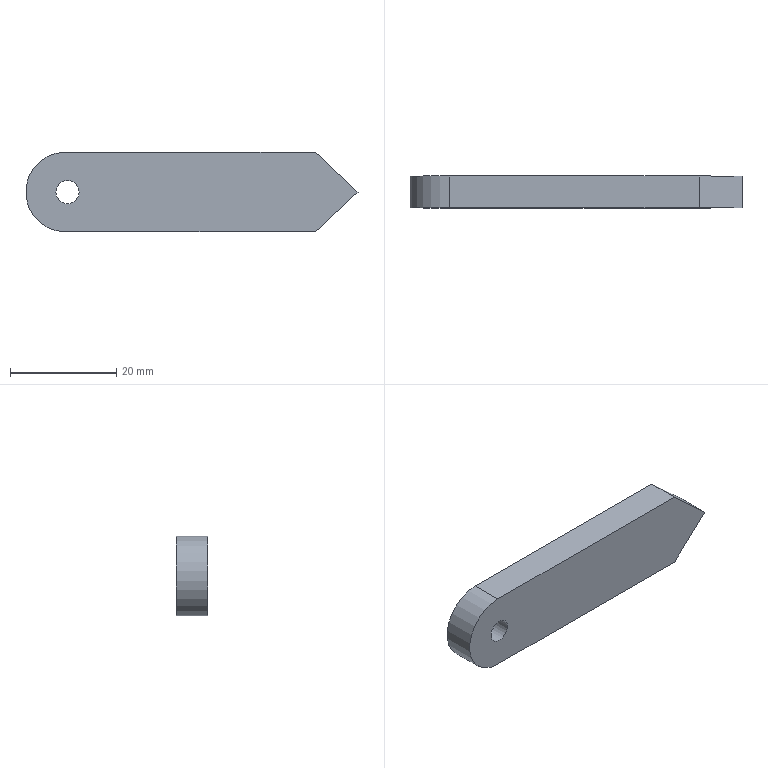Component | NX | TRI_SLIDER_2 | 1 solid | 8 faces | box 62.5 x 6 x 15 mm | volume 5028 mm3 | plane 6 | cylinder 2 | commonest cylinder face diameters 15 x1 4.371 x1
STEP:
#1=CARTESIAN_POINT('',(0.,0.,0.));
#2=DIRECTION('',(0.,0.,1.));
#3=DIRECTION('',(1.,0.,0.));
#4=AXIS2_PLACEMENT_3D('',#1,#2,#3);
#5=CARTESIAN_POINT('',(53.887,-12.,79.479));
#6=VERTEX_POINT('',#5);
#7=CARTESIAN_POINT('',(45.867,-12.,72.));
#8=VERTEX_POINT('',#7);
#9=CARTESIAN_POINT('',(53.887,-12.,79.479));
#10=DIRECTION('',(-0.7314,0.,-0.682));
#11=VECTOR('',#10,1.);
#12=LINE('',#9,#11);
#13=CARTESIAN_POINT('',(53.887,-18.,79.479));
#14=DIRECTION('',(0.682,0.,-0.7314));
#15=DIRECTION('',(0.7314,0.,0.682));
#16=AXIS2_PLACEMENT_3D('',#13,#14,#15);
#17=PLANE('',#16);
#18=CARTESIAN_POINT('',(0.,-6.));
#19=DIRECTION('',(-1.,0.));
#20=VECTOR('',#19,1.);
#21=LINE('',#18,#20);
#22=(GEOMETRIC_REPRESENTATION_CONTEXT(2)PARAMETRIC_REPRESENTATION_CONTEXT()REPRESENTATION_CONTEXT('',''));
#23=DEFINITIONAL_REPRESENTATION('',(#21),#22);
#24=PCURVE('',#17,#23);
#25=CARTESIAN_POINT('',(-1.113,-12.,79.5));
#26=DIRECTION('',(0.,1.,0.));
#27=DIRECTION('',(1.,0.,0.));
#28=AXIS2_PLACEMENT_3D('',#25,#26,#27);
#29=PLANE('',#28);
#30=CARTESIAN_POINT('',(55.,0.02132));
#31=DIRECTION('',(-0.7314,0.682));
#32=VECTOR('',#31,1.);
#33=LINE('',#30,#32);
#34=(GEOMETRIC_REPRESENTATION_CONTEXT(2)PARAMETRIC_REPRESENTATION_CONTEXT()REPRESENTATION_CONTEXT('',''));
#35=DEFINITIONAL_REPRESENTATION('',(#33),#34);
#36=PCURVE('',#29,#35);
#37=SURFACE_CURVE('',#12,(#24,#36),.PCURVE_S1.);
#38=EDGE_CURVE('',#6,#8,#37,.T.);
#39=ORIENTED_EDGE('',*,*,#38,.F.);
#40=CARTESIAN_POINT('',(53.887,-18.,79.479));
#41=VERTEX_POINT('',#40);
#42=CARTESIAN_POINT('',(53.887,-18.,79.479));
#43=DIRECTION('',(0.,1.,0.));
#44=VECTOR('',#43,1.);
#45=LINE('',#42,#44);
#46=CARTESIAN_POINT('',(0.,0.));
#47=DIRECTION('',(0.,-1.));
#48=VECTOR('',#47,1.);
#49=LINE('',#46,#48);
#50=(GEOMETRIC_REPRESENTATION_CONTEXT(2)PARAMETRIC_REPRESENTATION_CONTEXT()REPRESENTATION_CONTEXT('',''));
#51=DEFINITIONAL_REPRESENTATION('',(#49),#50);
#52=PCURVE('',#17,#51);
#53=CARTESIAN_POINT('',(45.822,-18.,87.));
#54=DIRECTION('',(0.682,0.,0.7314));
#55=DIRECTION('',(-0.7314,0.,0.682));
#56=AXIS2_PLACEMENT_3D('',#53,#54,#55);
#57=PLANE('',#56);
#58=CARTESIAN_POINT('',(-11.028,0.));
#59=DIRECTION('',(0.,-1.));
#60=VECTOR('',#59,1.);
#61=LINE('',#58,#60);
#62=(GEOMETRIC_REPRESENTATION_CONTEXT(2)PARAMETRIC_REPRESENTATION_CONTEXT()REPRESENTATION_CONTEXT('',''));
#63=DEFINITIONAL_REPRESENTATION('',(#61),#62);
#64=PCURVE('',#57,#63);
#65=SURFACE_CURVE('',#45,(#52,#64),.PCURVE_S1.);
#66=EDGE_CURVE('',#41,#6,#65,.T.);
#67=ORIENTED_EDGE('',*,*,#66,.F.);
#68=CARTESIAN_POINT('',(45.867,-18.,72.));
#69=VERTEX_POINT('',#68);
#70=CARTESIAN_POINT('',(53.887,-18.,79.479));
#71=DIRECTION('',(-0.7314,0.,-0.682));
#72=VECTOR('',#71,1.);
#73=LINE('',#70,#72);
#74=CARTESIAN_POINT('',(0.,0.));
#75=DIRECTION('',(-1.,0.));
#76=VECTOR('',#75,1.);
#77=LINE('',#74,#76);
#78=(GEOMETRIC_REPRESENTATION_CONTEXT(2)PARAMETRIC_REPRESENTATION_CONTEXT()REPRESENTATION_CONTEXT('',''));
#79=DEFINITIONAL_REPRESENTATION('',(#77),#78);
#80=PCURVE('',#17,#79);
#81=CARTESIAN_POINT('',(-1.113,-18.,79.5));
#82=DIRECTION('',(0.,1.,0.));
#83=DIRECTION('',(1.,0.,0.));
#84=AXIS2_PLACEMENT_3D('',#81,#82,#83);
#85=PLANE('',#84);
#86=CARTESIAN_POINT('',(55.,0.02132));
#87=DIRECTION('',(-0.7314,0.682));
#88=VECTOR('',#87,1.);
#89=LINE('',#86,#88);
#90=(GEOMETRIC_REPRESENTATION_CONTEXT(2)PARAMETRIC_REPRESENTATION_CONTEXT()REPRESENTATION_CONTEXT('',''));
#91=DEFINITIONAL_REPRESENTATION('',(#89),#90);
#92=PCURVE('',#85,#91);
#93=SURFACE_CURVE('',#73,(#80,#92),.PCURVE_S1.);
#94=EDGE_CURVE('',#41,#69,#93,.T.);
#95=ORIENTED_EDGE('',*,*,#94,.T.);
#96=CARTESIAN_POINT('',(45.867,-18.,72.));
#97=DIRECTION('',(0.,1.,0.));
#98=VECTOR('',#97,1.);
#99=LINE('',#96,#98);
#100=CARTESIAN_POINT('',(-10.966,0.));
#101=DIRECTION('',(0.,-1.));
#102=VECTOR('',#101,1.);
#103=LINE('',#100,#102);
#104=(GEOMETRIC_REPRESENTATION_CONTEXT(2)PARAMETRIC_REPRESENTATION_CONTEXT()REPRESENTATION_CONTEXT('',''));
#105=DEFINITIONAL_REPRESENTATION('',(#103),#104);
#106=PCURVE('',#17,#105);
#107=CARTESIAN_POINT('',(45.867,-18.,72.));
#108=DIRECTION('',(0.,0.,-1.));
#109=DIRECTION('',(1.,0.,0.));
#110=AXIS2_PLACEMENT_3D('',#107,#108,#109);
#111=PLANE('',#110);
#112=CARTESIAN_POINT('',(0.,0.));
#113=DIRECTION('',(0.,-1.));
#114=VECTOR('',#113,1.);
#115=LINE('',#112,#114);
#116=(GEOMETRIC_REPRESENTATION_CONTEXT(2)PARAMETRIC_REPRESENTATION_CONTEXT()REPRESENTATION_CONTEXT('',''));
#117=DEFINITIONAL_REPRESENTATION('',(#115),#116);
#118=PCURVE('',#111,#117);
#119=SURFACE_CURVE('',#99,(#106,#118),.PCURVE_S1.);
#120=EDGE_CURVE('',#69,#8,#119,.T.);
#121=ORIENTED_EDGE('',*,*,#120,.T.);
#122=EDGE_LOOP('',(#39,#67,#95,#121));
#123=FACE_BOUND('',#122,.T.);
#124=ADVANCED_FACE('',(#123),#17,.T.);
#125=CARTESIAN_POINT('',(-1.113,-12.,72.));
#126=VERTEX_POINT('',#125);
#127=CARTESIAN_POINT('',(45.867,-12.,72.));
#128=DIRECTION('',(-1.,0.,-0.));
#129=VECTOR('',#128,1.);
#130=LINE('',#127,#129);
#131=CARTESIAN_POINT('',(0.,-6.));
#132=DIRECTION('',(-1.,0.));
#133=VECTOR('',#132,1.);
#134=LINE('',#131,#133);
#135=(GEOMETRIC_REPRESENTATION_CONTEXT(2)PARAMETRIC_REPRESENTATION_CONTEXT()REPRESENTATION_CONTEXT('',''));
#136=DEFINITIONAL_REPRESENTATION('',(#134),#135);
#137=PCURVE('',#111,#136);
#138=CARTESIAN_POINT('',(46.98,7.5));
#139=DIRECTION('',(-1.,0.));
#140=VECTOR('',#139,1.);
#141=LINE('',#138,#140);
#142=(GEOMETRIC_REPRESENTATION_CONTEXT(2)PARAMETRIC_REPRESENTATION_CONTEXT()REPRESENTATION_CONTEXT('',''));
#143=DEFINITIONAL_REPRESENTATION('',(#141),#142);
#144=PCURVE('',#29,#143);
#145=SURFACE_CURVE('',#130,(#137,#144),.PCURVE_S1.);
#146=EDGE_CURVE('',#8,#126,#145,.T.);
#147=ORIENTED_EDGE('',*,*,#146,.F.);
#148=ORIENTED_EDGE('',*,*,#120,.F.);
#149=CARTESIAN_POINT('',(-1.113,-18.,72.));
#150=VERTEX_POINT('',#149);
#151=CARTESIAN_POINT('',(45.867,-18.,72.));
#152=DIRECTION('',(-1.,0.,-0.));
#153=VECTOR('',#152,1.);
#154=LINE('',#151,#153);
#155=CARTESIAN_POINT('',(0.,0.));
#156=DIRECTION('',(-1.,0.));
#157=VECTOR('',#156,1.);
#158=LINE('',#155,#157);
#159=(GEOMETRIC_REPRESENTATION_CONTEXT(2)PARAMETRIC_REPRESENTATION_CONTEXT()REPRESENTATION_CONTEXT('',''));
#160=DEFINITIONAL_REPRESENTATION('',(#158),#159);
#161=PCURVE('',#111,#160);
#162=CARTESIAN_POINT('',(46.98,7.5));
#163=DIRECTION('',(-1.,0.));
#164=VECTOR('',#163,1.);
#165=LINE('',#162,#164);
#166=(GEOMETRIC_REPRESENTATION_CONTEXT(2)PARAMETRIC_REPRESENTATION_CONTEXT()REPRESENTATION_CONTEXT('',''));
#167=DEFINITIONAL_REPRESENTATION('',(#165),#166);
#168=PCURVE('',#85,#167);
#169=SURFACE_CURVE('',#154,(#161,#168),.PCURVE_S1.);
#170=EDGE_CURVE('',#69,#150,#169,.T.);
#171=ORIENTED_EDGE('',*,*,#170,.T.);
#172=CARTESIAN_POINT('',(-1.113,-18.,72.));
#173=DIRECTION('',(0.,1.,0.));
#174=VECTOR('',#173,1.);
#175=LINE('',#172,#174);
#176=CARTESIAN_POINT('',(-46.98,0.));
#177=DIRECTION('',(0.,-1.));
#178=VECTOR('',#177,1.);
#179=LINE('',#176,#178);
#180=(GEOMETRIC_REPRESENTATION_CONTEXT(2)PARAMETRIC_REPRESENTATION_CONTEXT()REPRESENTATION_CONTEXT('',''));
#181=DEFINITIONAL_REPRESENTATION('',(#179),#180);
#182=PCURVE('',#111,#181);
#183=CARTESIAN_POINT('',(-1.113,-18.,79.5));
#184=DIRECTION('',(0.,1.,0.));
#185=DIRECTION('',(1.,0.,0.));
#186=AXIS2_PLACEMENT_3D('',#183,#184,#185);
#187=CYLINDRICAL_SURFACE('',#186,7.5);
#188=CARTESIAN_POINT('',(1.571,0.));
#189=DIRECTION('',(0.,1.));
#190=VECTOR('',#189,1.);
#191=LINE('',#188,#190);
#192=(GEOMETRIC_REPRESENTATION_CONTEXT(2)PARAMETRIC_REPRESENTATION_CONTEXT()REPRESENTATION_CONTEXT('',''));
#193=DEFINITIONAL_REPRESENTATION('',(#191),#192);
#194=PCURVE('',#187,#193);
#195=SURFACE_CURVE('',#175,(#182,#194),.PCURVE_S1.);
#196=EDGE_CURVE('',#150,#126,#195,.T.);
#197=ORIENTED_EDGE('',*,*,#196,.T.);
#198=EDGE_LOOP('',(#147,#148,#171,#197));
#199=FACE_BOUND('',#198,.T.);
#200=ADVANCED_FACE('',(#199),#111,.T.);
#201=CARTESIAN_POINT('',(-1.113,-12.,87.));
#202=VERTEX_POINT('',#201);
#203=CARTESIAN_POINT('',(-1.113,-12.,79.5));
#204=DIRECTION('',(0.,1.,0.));
#205=DIRECTION('',(-1.,0.,0.));
#206=AXIS2_PLACEMENT_3D('',#203,#204,#205);
#207=CIRCLE('',#206,7.5);
#208=CARTESIAN_POINT('',(-3.142,6.));
#209=DIRECTION('',(1.,0.));
#210=VECTOR('',#209,1.);
#211=LINE('',#208,#210);
#212=(GEOMETRIC_REPRESENTATION_CONTEXT(2)PARAMETRIC_REPRESENTATION_CONTEXT()REPRESENTATION_CONTEXT('',''));
#213=DEFINITIONAL_REPRESENTATION('',(#211),#212);
#214=PCURVE('',#187,#213);
#215=CARTESIAN_POINT('',(0.,0.));
#216=DIRECTION('',(-1.,0.));
#217=AXIS2_PLACEMENT_2D('',#215,#216);
#218=CIRCLE('',#217,7.5);
#219=(GEOMETRIC_REPRESENTATION_CONTEXT(2)PARAMETRIC_REPRESENTATION_CONTEXT()REPRESENTATION_CONTEXT('',''));
#220=DEFINITIONAL_REPRESENTATION('',(#218),#219);
#221=PCURVE('',#29,#220);
#222=SURFACE_CURVE('',#207,(#214,#221),.PCURVE_S1.);
#223=EDGE_CURVE('',#126,#202,#222,.T.);
#224=ORIENTED_EDGE('',*,*,#223,.F.);
#225=ORIENTED_EDGE('',*,*,#196,.F.);
#226=CARTESIAN_POINT('',(-1.113,-18.,87.));
#227=VERTEX_POINT('',#226);
#228=CARTESIAN_POINT('',(-1.113,-18.,79.5));
#229=DIRECTION('',(0.,1.,0.));
#230=DIRECTION('',(-1.,0.,0.));
#231=AXIS2_PLACEMENT_3D('',#228,#229,#230);
#232=CIRCLE('',#231,7.5);
#233=CARTESIAN_POINT('',(-3.142,0.));
#234=DIRECTION('',(1.,0.));
#235=VECTOR('',#234,1.);
#236=LINE('',#233,#235);
#237=(GEOMETRIC_REPRESENTATION_CONTEXT(2)PARAMETRIC_REPRESENTATION_CONTEXT()REPRESENTATION_CONTEXT('',''));
#238=DEFINITIONAL_REPRESENTATION('',(#236),#237);
#239=PCURVE('',#187,#238);
#240=CARTESIAN_POINT('',(0.,0.));
#241=DIRECTION('',(-1.,0.));
#242=AXIS2_PLACEMENT_2D('',#240,#241);
#243=CIRCLE('',#242,7.5);
#244=(GEOMETRIC_REPRESENTATION_CONTEXT(2)PARAMETRIC_REPRESENTATION_CONTEXT()REPRESENTATION_CONTEXT('',''));
#245=DEFINITIONAL_REPRESENTATION('',(#243),#244);
#246=PCURVE('',#85,#245);
#247=SURFACE_CURVE('',#232,(#239,#246),.PCURVE_S1.);
#248=EDGE_CURVE('',#150,#227,#247,.T.);
#249=ORIENTED_EDGE('',*,*,#248,.T.);
#250=CARTESIAN_POINT('',(-1.113,-18.,87.));
#251=DIRECTION('',(0.,1.,0.));
#252=VECTOR('',#251,1.);
#253=LINE('',#250,#252);
#254=CARTESIAN_POINT('',(4.712,0.));
#255=DIRECTION('',(0.,1.));
#256=VECTOR('',#255,1.);
#257=LINE('',#254,#256);
#258=(GEOMETRIC_REPRESENTATION_CONTEXT(2)PARAMETRIC_REPRESENTATION_CONTEXT()REPRESENTATION_CONTEXT('',''));
#259=DEFINITIONAL_REPRESENTATION('',(#257),#258);
#260=PCURVE('',#187,#259);
#261=CARTESIAN_POINT('',(-1.113,-18.,87.));
#262=DIRECTION('',(-0.,0.,1.));
#263=DIRECTION('',(-1.,0.,-0.));
#264=AXIS2_PLACEMENT_3D('',#261,#262,#263);
#265=PLANE('',#264);
#266=CARTESIAN_POINT('',(0.,0.));
#267=DIRECTION('',(0.,-1.));
#268=VECTOR('',#267,1.);
#269=LINE('',#266,#268);
#270=(GEOMETRIC_REPRESENTATION_CONTEXT(2)PARAMETRIC_REPRESENTATION_CONTEXT()REPRESENTATION_CONTEXT('',''));
#271=DEFINITIONAL_REPRESENTATION('',(#269),#270);
#272=PCURVE('',#265,#271);
#273=SURFACE_CURVE('',#253,(#260,#272),.PCURVE_S1.);
#274=EDGE_CURVE('',#227,#202,#273,.T.);
#275=ORIENTED_EDGE('',*,*,#274,.T.);
#276=EDGE_LOOP('',(#224,#225,#249,#275));
#277=FACE_BOUND('',#276,.T.);
#278=ADVANCED_FACE('',(#277),#187,.T.);
#279=CARTESIAN_POINT('',(45.822,-12.,87.));
#280=VERTEX_POINT('',#279);
#281=CARTESIAN_POINT('',(-1.113,-12.,87.));
#282=DIRECTION('',(1.,0.,0.));
#283=VECTOR('',#282,1.);
#284=LINE('',#281,#283);
#285=CARTESIAN_POINT('',(0.,-6.));
#286=DIRECTION('',(-1.,0.));
#287=VECTOR('',#286,1.);
#288=LINE('',#285,#287);
#289=(GEOMETRIC_REPRESENTATION_CONTEXT(2)PARAMETRIC_REPRESENTATION_CONTEXT()REPRESENTATION_CONTEXT('',''));
#290=DEFINITIONAL_REPRESENTATION('',(#288),#289);
#291=PCURVE('',#265,#290);
#292=CARTESIAN_POINT('',(0.,-7.5));
#293=DIRECTION('',(1.,-0.));
#294=VECTOR('',#293,1.);
#295=LINE('',#292,#294);
#296=(GEOMETRIC_REPRESENTATION_CONTEXT(2)PARAMETRIC_REPRESENTATION_CONTEXT()REPRESENTATION_CONTEXT('',''));
#297=DEFINITIONAL_REPRESENTATION('',(#295),#296);
#298=PCURVE('',#29,#297);
#299=SURFACE_CURVE('',#284,(#291,#298),.PCURVE_S1.);
#300=EDGE_CURVE('',#202,#280,#299,.T.);
#301=ORIENTED_EDGE('',*,*,#300,.F.);
#302=ORIENTED_EDGE('',*,*,#274,.F.);
#303=CARTESIAN_POINT('',(45.822,-18.,87.));
#304=VERTEX_POINT('',#303);
#305=CARTESIAN_POINT('',(-1.113,-18.,87.));
#306=DIRECTION('',(1.,0.,0.));
#307=VECTOR('',#306,1.);
#308=LINE('',#305,#307);
#309=CARTESIAN_POINT('',(0.,0.));
#310=DIRECTION('',(-1.,0.));
#311=VECTOR('',#310,1.);
#312=LINE('',#309,#311);
#313=(GEOMETRIC_REPRESENTATION_CONTEXT(2)PARAMETRIC_REPRESENTATION_CONTEXT()REPRESENTATION_CONTEXT('',''));
#314=DEFINITIONAL_REPRESENTATION('',(#312),#313);
#315=PCURVE('',#265,#314);
#316=CARTESIAN_POINT('',(0.,-7.5));
#317=DIRECTION('',(1.,-0.));
#318=VECTOR('',#317,1.);
#319=LINE('',#316,#318);
#320=(GEOMETRIC_REPRESENTATION_CONTEXT(2)PARAMETRIC_REPRESENTATION_CONTEXT()REPRESENTATION_CONTEXT('',''));
#321=DEFINITIONAL_REPRESENTATION('',(#319),#320);
#322=PCURVE('',#85,#321);
#323=SURFACE_CURVE('',#308,(#315,#322),.PCURVE_S1.);
#324=EDGE_CURVE('',#227,#304,#323,.T.);
#325=ORIENTED_EDGE('',*,*,#324,.T.);
#326=CARTESIAN_POINT('',(45.822,-18.,87.));
#327=DIRECTION('',(0.,1.,0.));
#328=VECTOR('',#327,1.);
#329=LINE('',#326,#328);
#330=CARTESIAN_POINT('',(-46.934,0.));
#331=DIRECTION('',(0.,-1.));
#332=VECTOR('',#331,1.);
#333=LINE('',#330,#332);
#334=(GEOMETRIC_REPRESENTATION_CONTEXT(2)PARAMETRIC_REPRESENTATION_CONTEXT()REPRESENTATION_CONTEXT('',''));
#335=DEFINITIONAL_REPRESENTATION('',(#333),#334);
#336=PCURVE('',#265,#335);
#337=CARTESIAN_POINT('',(0.,0.));
#338=DIRECTION('',(0.,-1.));
#339=VECTOR('',#338,1.);
#340=LINE('',#337,#339);
#341=(GEOMETRIC_REPRESENTATION_CONTEXT(2)PARAMETRIC_REPRESENTATION_CONTEXT()REPRESENTATION_CONTEXT('',''));
#342=DEFINITIONAL_REPRESENTATION('',(#340),#341);
#343=PCURVE('',#57,#342);
#344=SURFACE_CURVE('',#329,(#336,#343),.PCURVE_S1.);
#345=EDGE_CURVE('',#304,#280,#344,.T.);
#346=ORIENTED_EDGE('',*,*,#345,.T.);
#347=EDGE_LOOP('',(#301,#302,#325,#346));
#348=FACE_BOUND('',#347,.T.);
#349=ADVANCED_FACE('',(#348),#265,.T.);
#350=CARTESIAN_POINT('',(45.822,-12.,87.));
#351=DIRECTION('',(0.7314,0.,-0.682));
#352=VECTOR('',#351,1.);
#353=LINE('',#350,#352);
#354=CARTESIAN_POINT('',(0.,-6.));
#355=DIRECTION('',(-1.,0.));
#356=VECTOR('',#355,1.);
#357=LINE('',#354,#356);
#358=(GEOMETRIC_REPRESENTATION_CONTEXT(2)PARAMETRIC_REPRESENTATION_CONTEXT()REPRESENTATION_CONTEXT('',''));
#359=DEFINITIONAL_REPRESENTATION('',(#357),#358);
#360=PCURVE('',#57,#359);
#361=CARTESIAN_POINT('',(46.934,-7.5));
#362=DIRECTION('',(0.7314,0.682));
#363=VECTOR('',#362,1.);
#364=LINE('',#361,#363);
#365=(GEOMETRIC_REPRESENTATION_CONTEXT(2)PARAMETRIC_REPRESENTATION_CONTEXT()REPRESENTATION_CONTEXT('',''));
#366=DEFINITIONAL_REPRESENTATION('',(#364),#365);
#367=PCURVE('',#29,#366);
#368=SURFACE_CURVE('',#353,(#360,#367),.PCURVE_S1.);
#369=EDGE_CURVE('',#280,#6,#368,.T.);
#370=ORIENTED_EDGE('',*,*,#369,.F.);
#371=ORIENTED_EDGE('',*,*,#345,.F.);
#372=CARTESIAN_POINT('',(45.822,-18.,87.));
#373=DIRECTION('',(0.7314,0.,-0.682));
#374=VECTOR('',#373,1.);
#375=LINE('',#372,#374);
#376=CARTESIAN_POINT('',(0.,0.));
#377=DIRECTION('',(-1.,0.));
#378=VECTOR('',#377,1.);
#379=LINE('',#376,#378);
#380=(GEOMETRIC_REPRESENTATION_CONTEXT(2)PARAMETRIC_REPRESENTATION_CONTEXT()REPRESENTATION_CONTEXT('',''));
#381=DEFINITIONAL_REPRESENTATION('',(#379),#380);
#382=PCURVE('',#57,#381);
#383=CARTESIAN_POINT('',(46.934,-7.5));
#384=DIRECTION('',(0.7314,0.682));
#385=VECTOR('',#384,1.);
#386=LINE('',#383,#385);
#387=(GEOMETRIC_REPRESENTATION_CONTEXT(2)PARAMETRIC_REPRESENTATION_CONTEXT()REPRESENTATION_CONTEXT('',''));
#388=DEFINITIONAL_REPRESENTATION('',(#386),#387);
#389=PCURVE('',#85,#388);
#390=SURFACE_CURVE('',#375,(#382,#389),.PCURVE_S1.);
#391=EDGE_CURVE('',#304,#41,#390,.T.);
#392=ORIENTED_EDGE('',*,*,#391,.T.);
#393=ORIENTED_EDGE('',*,*,#66,.T.);
#394=EDGE_LOOP('',(#370,#371,#392,#393));
#395=FACE_BOUND('',#394,.T.);
#396=ADVANCED_FACE('',(#395),#57,.T.);
#397=CARTESIAN_POINT('',(-2.938,-18.,79.479));
#398=VERTEX_POINT('',#397);
#399=CARTESIAN_POINT('',(-0.7529,-18.,79.479));
#400=DIRECTION('',(0.,-1.,0.));
#401=DIRECTION('',(-1.,0.,0.));
#402=AXIS2_PLACEMENT_3D('',#399,#400,#401);
#403=CIRCLE('',#402,2.186);
#404=CARTESIAN_POINT('',(-0.7529,-18.,79.479));
#405=DIRECTION('',(0.,1.,0.));
#406=DIRECTION('',(1.,0.,0.));
#407=AXIS2_PLACEMENT_3D('',#404,#405,#406);
#408=CYLINDRICAL_SURFACE('',#407,2.186);
#409=CARTESIAN_POINT('',(9.425,0.));
#410=DIRECTION('',(-1.,0.));
#411=VECTOR('',#410,1.);
#412=LINE('',#409,#411);
#413=(GEOMETRIC_REPRESENTATION_CONTEXT(2)PARAMETRIC_REPRESENTATION_CONTEXT()REPRESENTATION_CONTEXT('',''));
#414=DEFINITIONAL_REPRESENTATION('',(#412),#413);
#415=PCURVE('',#408,#414);
#416=CARTESIAN_POINT('',(-1.826,0.02132));
#417=CARTESIAN_POINT('',(-1.826,3.807));
#418=CARTESIAN_POINT('',(1.453,1.914));
#419=CARTESIAN_POINT('',(4.731,0.02132));
#420=CARTESIAN_POINT('',(1.453,-1.871));
#421=CARTESIAN_POINT('',(-1.826,-3.764));
#422=CARTESIAN_POINT('',(-1.826,0.02132));
#423=(BOUNDED_CURVE()B_SPLINE_CURVE(2,(#416,#417,#418,#419,#420,#421,#422),.UNSPECIFIED.,.T.,.F.)B_SPLINE_CURVE_WITH_KNOTS((1,2,2,2,2,1),(-2.094,0.,2.094,4.189,6.283,8.378),.UNSPECIFIED.)CURVE()GEOMETRIC_REPRESENTATION_ITEM()RATIONAL_B_SPLINE_CURVE((1.,0.5,1.,0.5,1.,0.5,1.))REPRESENTATION_ITEM(''));
#424=(GEOMETRIC_REPRESENTATION_CONTEXT(2)PARAMETRIC_REPRESENTATION_CONTEXT()REPRESENTATION_CONTEXT('',''));
#425=DEFINITIONAL_REPRESENTATION('',(#423),#424);
#426=PCURVE('',#85,#425);
#427=SURFACE_CURVE('',#403,(#415,#426),.PCURVE_S1.);
#428=EDGE_CURVE('',#398,#398,#427,.T.);
#429=ORIENTED_EDGE('',*,*,#428,.F.);
#430=CARTESIAN_POINT('',(-2.938,-12.,79.479));
#431=VERTEX_POINT('',#430);
#432=CARTESIAN_POINT('',(-2.938,-18.,79.479));
#433=CARTESIAN_POINT('',(-2.938,-12.,79.479));
#434=B_SPLINE_CURVE_WITH_KNOTS('',1,(#432,#433),.UNSPECIFIED.,.F.,.F.,(2,2),(0.,6.),.PIECEWISE_BEZIER_KNOTS.);
#435=CARTESIAN_POINT('',(9.425,0.));
#436=DIRECTION('',(0.,1.));
#437=VECTOR('',#436,1.);
#438=LINE('',#435,#437);
#439=(GEOMETRIC_REPRESENTATION_CONTEXT(2)PARAMETRIC_REPRESENTATION_CONTEXT()REPRESENTATION_CONTEXT('',''));
#440=DEFINITIONAL_REPRESENTATION('',(#438),#439);
#441=PCURVE('',#408,#440);
#442=CARTESIAN_POINT('',(3.142,0.));
#443=DIRECTION('',(0.,1.));
#444=VECTOR('',#443,1.);
#445=LINE('',#442,#444);
#446=(GEOMETRIC_REPRESENTATION_CONTEXT(2)PARAMETRIC_REPRESENTATION_CONTEXT()REPRESENTATION_CONTEXT('',''));
#447=DEFINITIONAL_REPRESENTATION('',(#445),#446);
#448=PCURVE('',#408,#447);
#449=SEAM_CURVE('',#434,(#441,#448),.PCURVE_S1.);
#450=EDGE_CURVE('',#398,#431,#449,.T.);
#451=ORIENTED_EDGE('',*,*,#450,.T.);
#452=CARTESIAN_POINT('',(-0.7529,-12.,79.479));
#453=DIRECTION('',(0.,-1.,0.));
#454=DIRECTION('',(-1.,0.,0.));
#455=AXIS2_PLACEMENT_3D('',#452,#453,#454);
#456=CIRCLE('',#455,2.186);
#457=CARTESIAN_POINT('',(9.425,6.));
#458=DIRECTION('',(-1.,0.));
#459=VECTOR('',#458,1.);
#460=LINE('',#457,#459);
#461=(GEOMETRIC_REPRESENTATION_CONTEXT(2)PARAMETRIC_REPRESENTATION_CONTEXT()REPRESENTATION_CONTEXT('',''));
#462=DEFINITIONAL_REPRESENTATION('',(#460),#461);
#463=PCURVE('',#408,#462);
#464=CARTESIAN_POINT('',(-1.826,0.02132));
#465=CARTESIAN_POINT('',(-1.826,3.807));
#466=CARTESIAN_POINT('',(1.453,1.914));
#467=CARTESIAN_POINT('',(4.731,0.02132));
#468=CARTESIAN_POINT('',(1.453,-1.871));
#469=CARTESIAN_POINT('',(-1.826,-3.764));
#470=CARTESIAN_POINT('',(-1.826,0.02132));
#471=(BOUNDED_CURVE()B_SPLINE_CURVE(2,(#464,#465,#466,#467,#468,#469,#470),.UNSPECIFIED.,.T.,.F.)B_SPLINE_CURVE_WITH_KNOTS((1,2,2,2,2,1),(-2.094,0.,2.094,4.189,6.283,8.378),.UNSPECIFIED.)CURVE()GEOMETRIC_REPRESENTATION_ITEM()RATIONAL_B_SPLINE_CURVE((1.,0.5,1.,0.5,1.,0.5,1.))REPRESENTATION_ITEM(''));
#472=(GEOMETRIC_REPRESENTATION_CONTEXT(2)PARAMETRIC_REPRESENTATION_CONTEXT()REPRESENTATION_CONTEXT('',''));
#473=DEFINITIONAL_REPRESENTATION('',(#471),#472);
#474=PCURVE('',#29,#473);
#475=SURFACE_CURVE('',#456,(#463,#474),.PCURVE_S1.);
#476=EDGE_CURVE('',#431,#431,#475,.T.);
#477=ORIENTED_EDGE('',*,*,#476,.T.);
#478=ORIENTED_EDGE('',*,*,#450,.F.);
#479=EDGE_LOOP('',(#429,#451,#477,#478));
#480=FACE_BOUND('',#479,.F.);
#481=ADVANCED_FACE('',(#480),#408,.F.);
#482=ORIENTED_EDGE('',*,*,#94,.F.);
#483=ORIENTED_EDGE('',*,*,#391,.F.);
#484=ORIENTED_EDGE('',*,*,#324,.F.);
#485=ORIENTED_EDGE('',*,*,#248,.F.);
#486=ORIENTED_EDGE('',*,*,#170,.F.);
#487=EDGE_LOOP('',(#482,#483,#484,#485,#486));
#488=FACE_BOUND('',#487,.T.);
#489=ORIENTED_EDGE('',*,*,#428,.F.);
#490=EDGE_LOOP('',(#489));
#491=FACE_BOUND('',#490,.T.);
#492=ADVANCED_FACE('',(#488,#491),#85,.F.);
#493=ORIENTED_EDGE('',*,*,#38,.T.);
#494=ORIENTED_EDGE('',*,*,#146,.T.);
#495=ORIENTED_EDGE('',*,*,#223,.T.);
#496=ORIENTED_EDGE('',*,*,#300,.T.);
#497=ORIENTED_EDGE('',*,*,#369,.T.);
#498=EDGE_LOOP('',(#493,#494,#495,#496,#497));
#499=FACE_BOUND('',#498,.T.);
#500=ORIENTED_EDGE('',*,*,#476,.T.);
#501=EDGE_LOOP('',(#500));
#502=FACE_BOUND('',#501,.T.);
#503=ADVANCED_FACE('',(#499,#502),#29,.T.);
#504=CLOSED_SHELL('',(#124,#200,#278,#349,#396,#481,#492,#503));
#505=MANIFOLD_SOLID_BREP('',#504);
#506=(LENGTH_UNIT()NAMED_UNIT(*)SI_UNIT(.MILLI.,.METRE.));
#507=UNCERTAINTY_MEASURE_WITH_UNIT(LENGTH_MEASURE(0.000001),#506,'','');
#508=(NAMED_UNIT(*)PLANE_ANGLE_UNIT()SI_UNIT($,.RADIAN.));
#509=(NAMED_UNIT(*)SI_UNIT($,.STERADIAN.)SOLID_ANGLE_UNIT());
#510=(GEOMETRIC_REPRESENTATION_CONTEXT(3)GLOBAL_UNCERTAINTY_ASSIGNED_CONTEXT((#507))GLOBAL_UNIT_ASSIGNED_CONTEXT((#506,#508,#509))REPRESENTATION_CONTEXT('',''));
#511=ADVANCED_BREP_SHAPE_REPRESENTATION('',(#4,#505),#510);